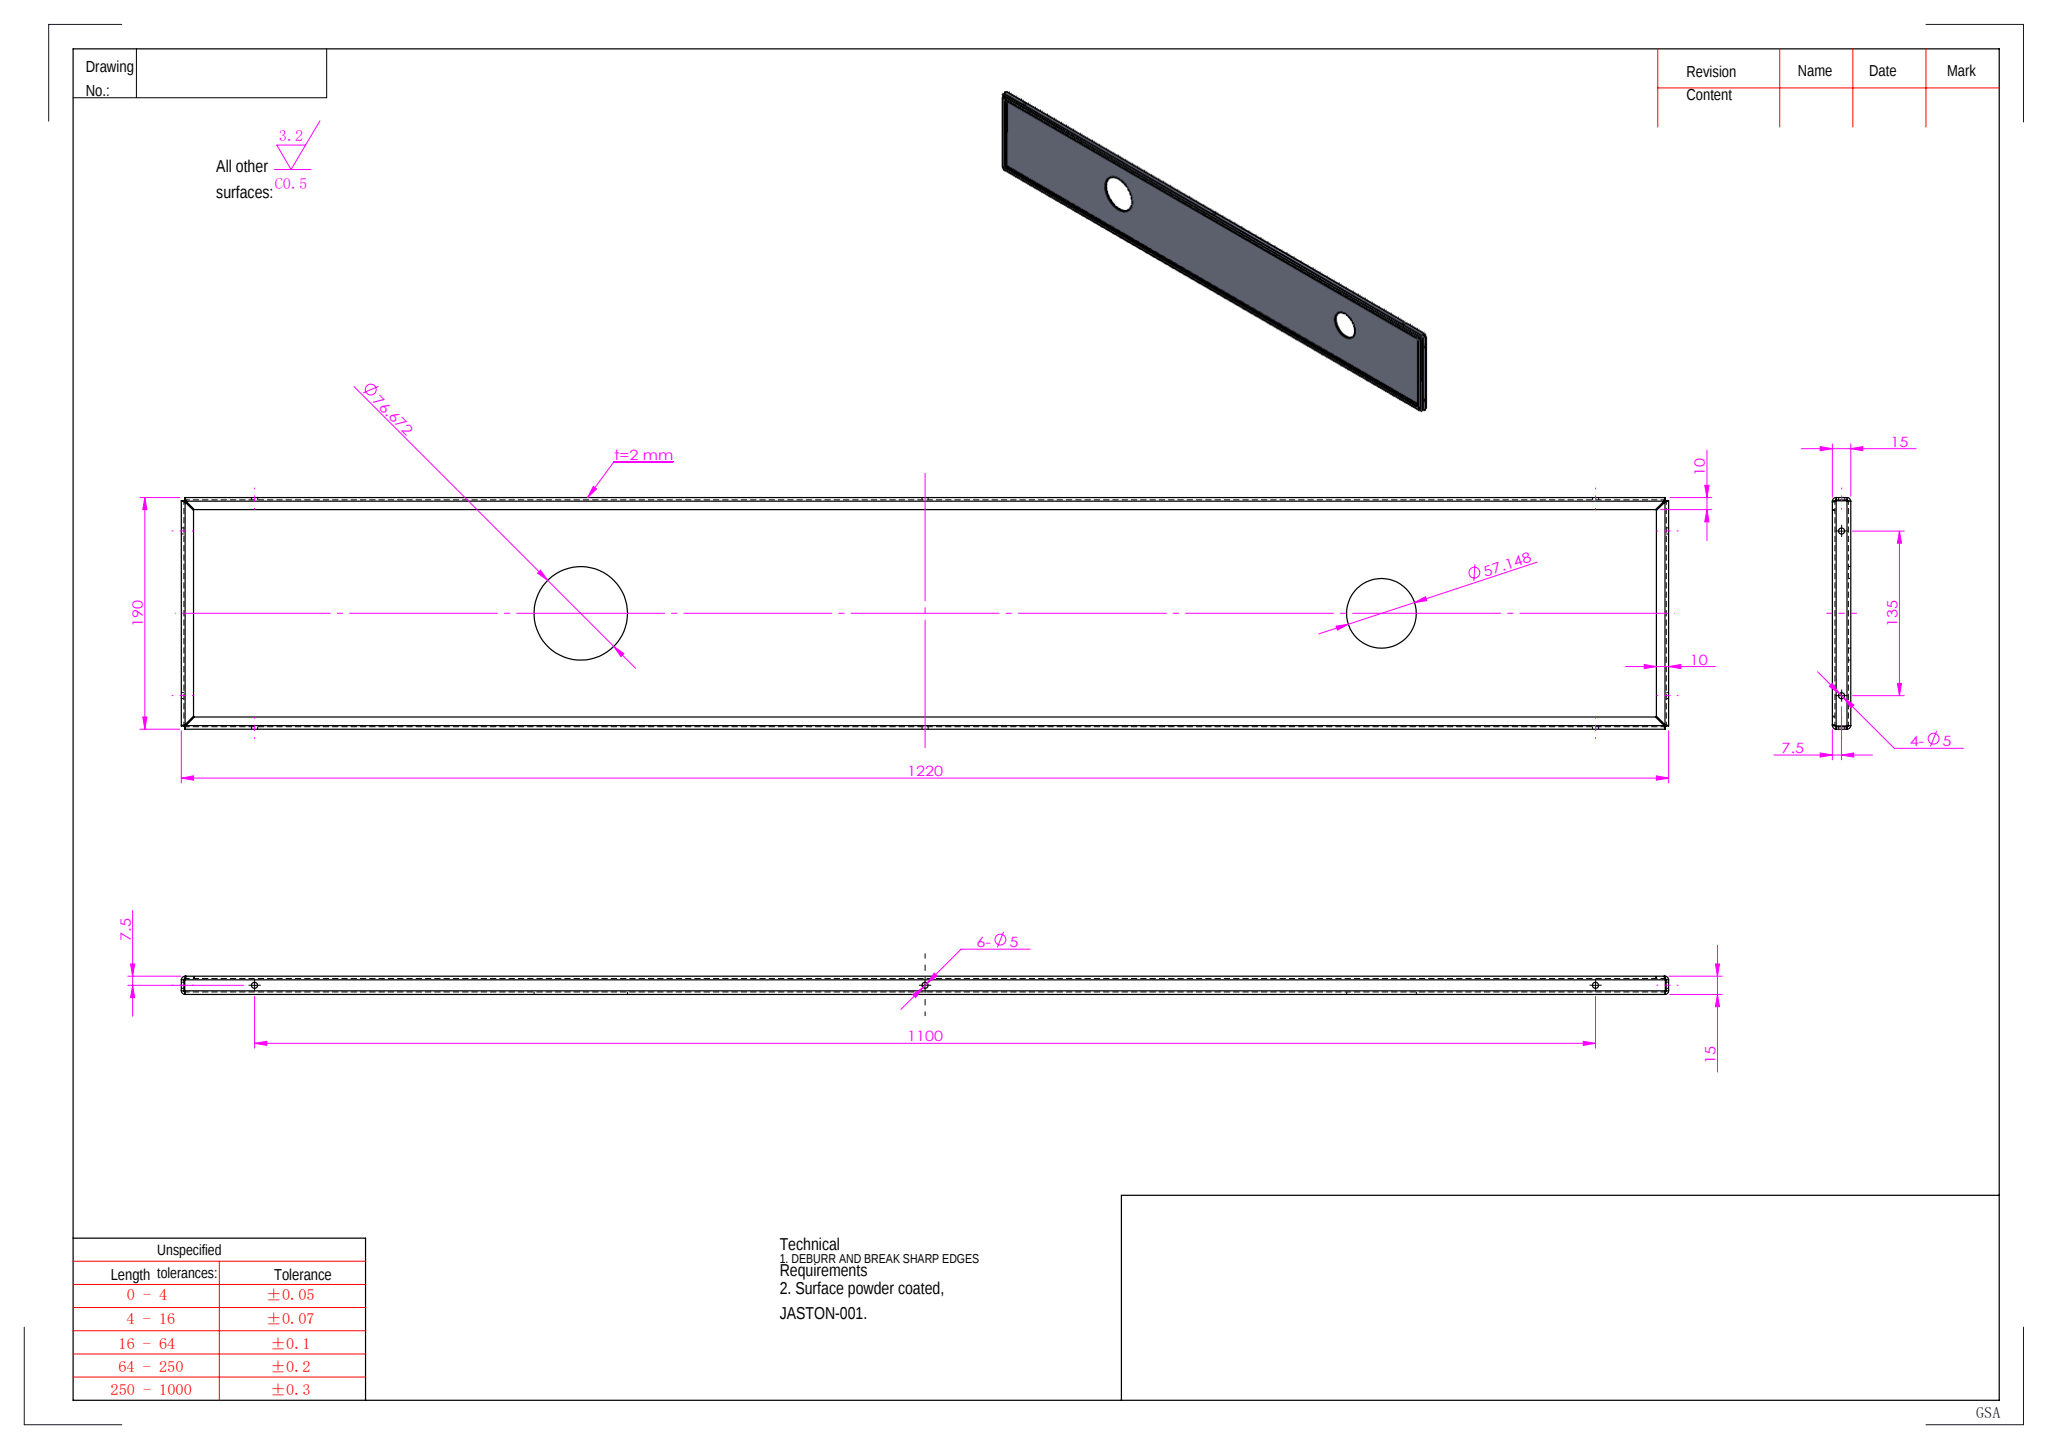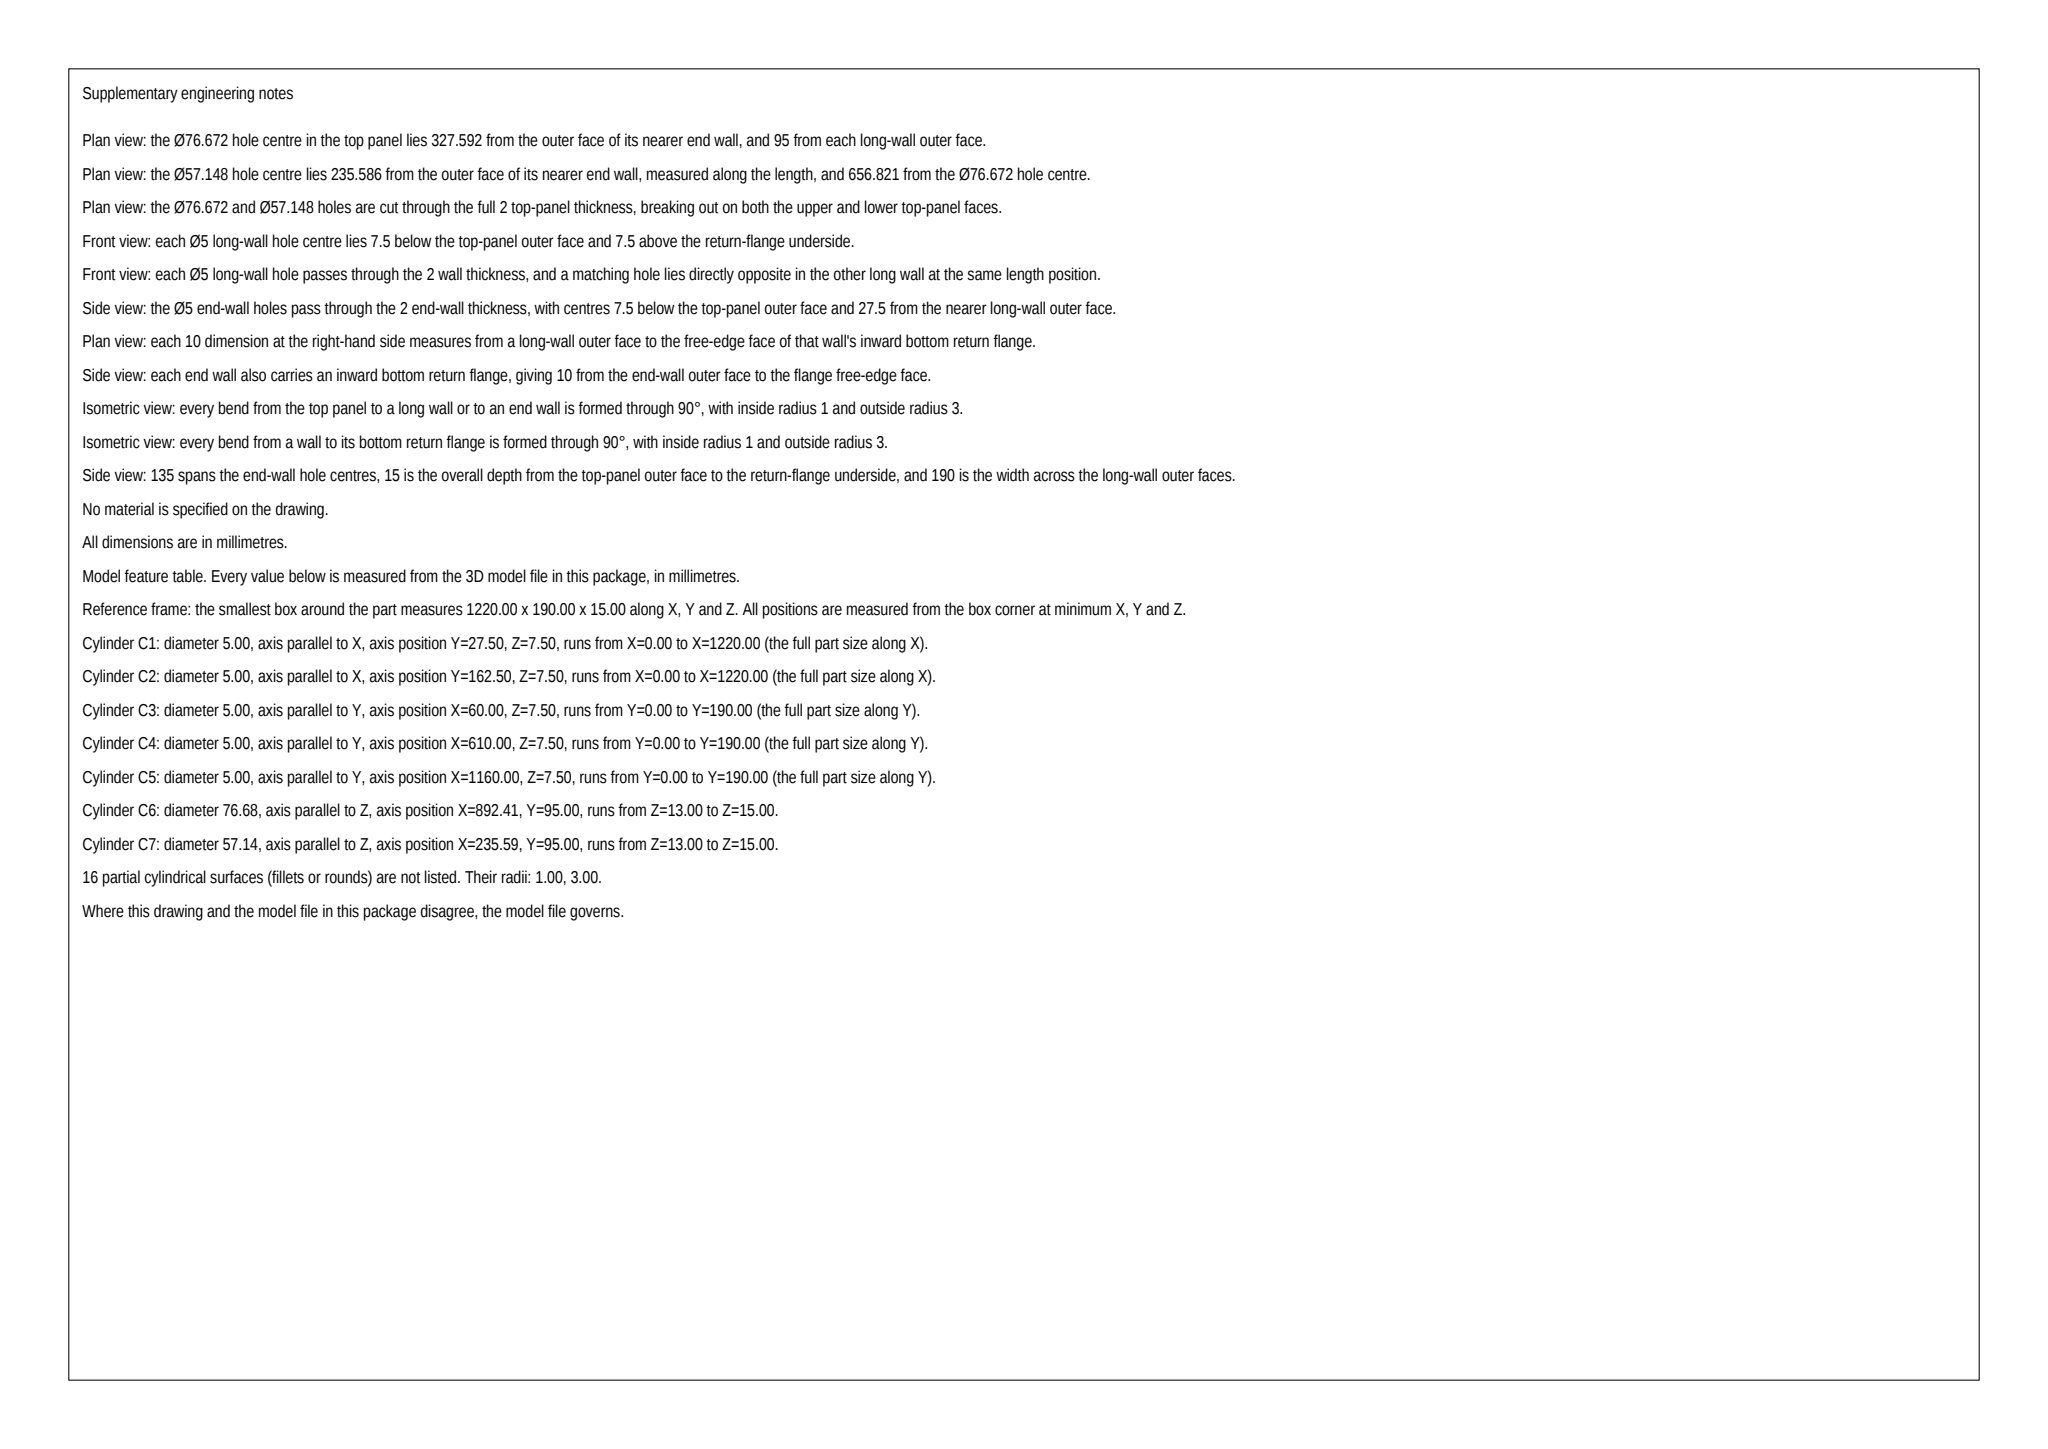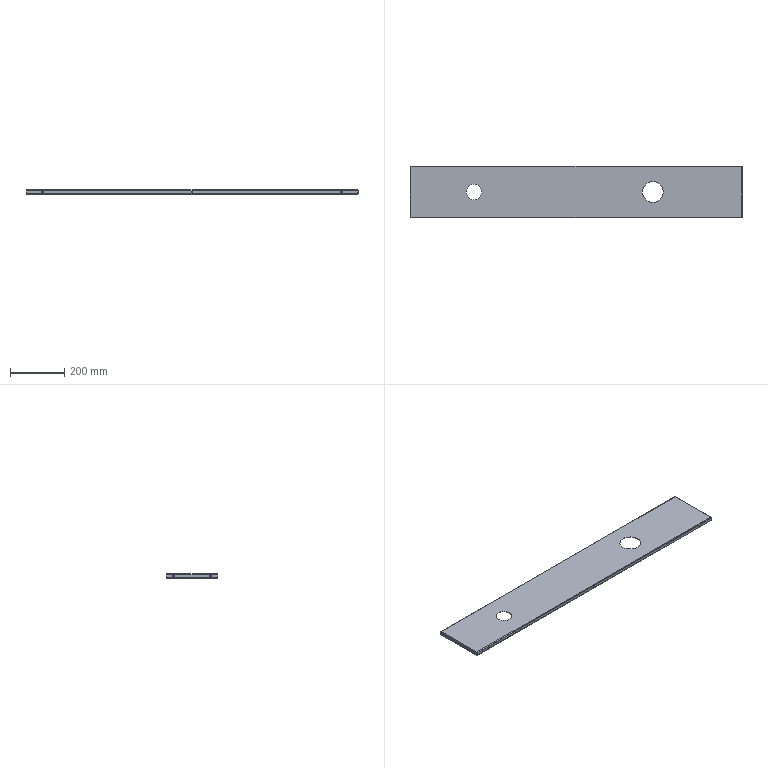Part | SolidWorks | mm | 1 solid | 94 faces | box 1220 x 190 x 15 mm | volume 556171 mm3 | cylinder 40 | plane 38 | spline 16 | commonest cylinder face diameters 5 x20 6 x8 2 x8 57.148 x2 76.672 x2